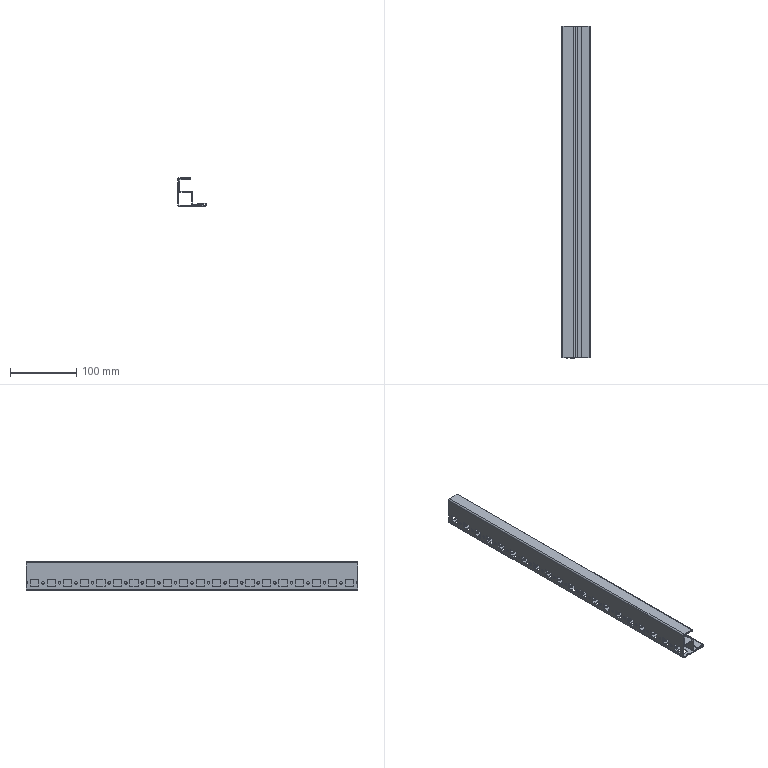Component | SolidWorks | CabinetFrameWeldmentDrawingPG50-01-00-1_LeftAndRightCrossBeamPG50-01-106-4 | 1 solid | 291 faces | volume 144431 mm3 | plane 188 | cylinder 103 | commonest cylinder face diameters 4.1 x85 1 x8 3.999 x6 4 x2 0.02 x1 3 x1 | material AISI 1045 Steel, cold drawn